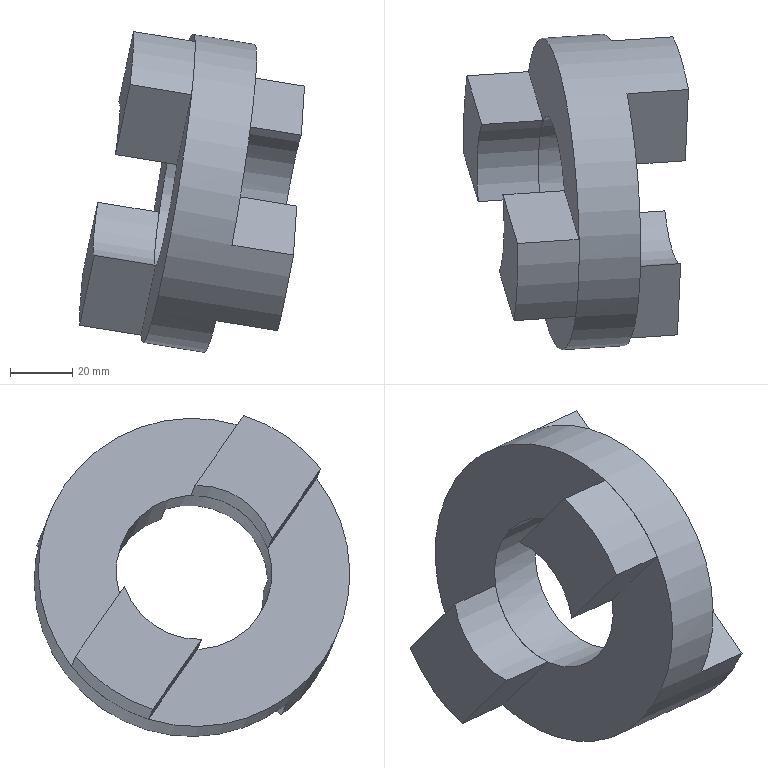Component | NX | 3 | 3 solids | 23 faces | volume 179810 mm3 | plane 17 | cylinder 6 | commonest cylinder face diameters 50 x3 100 x3